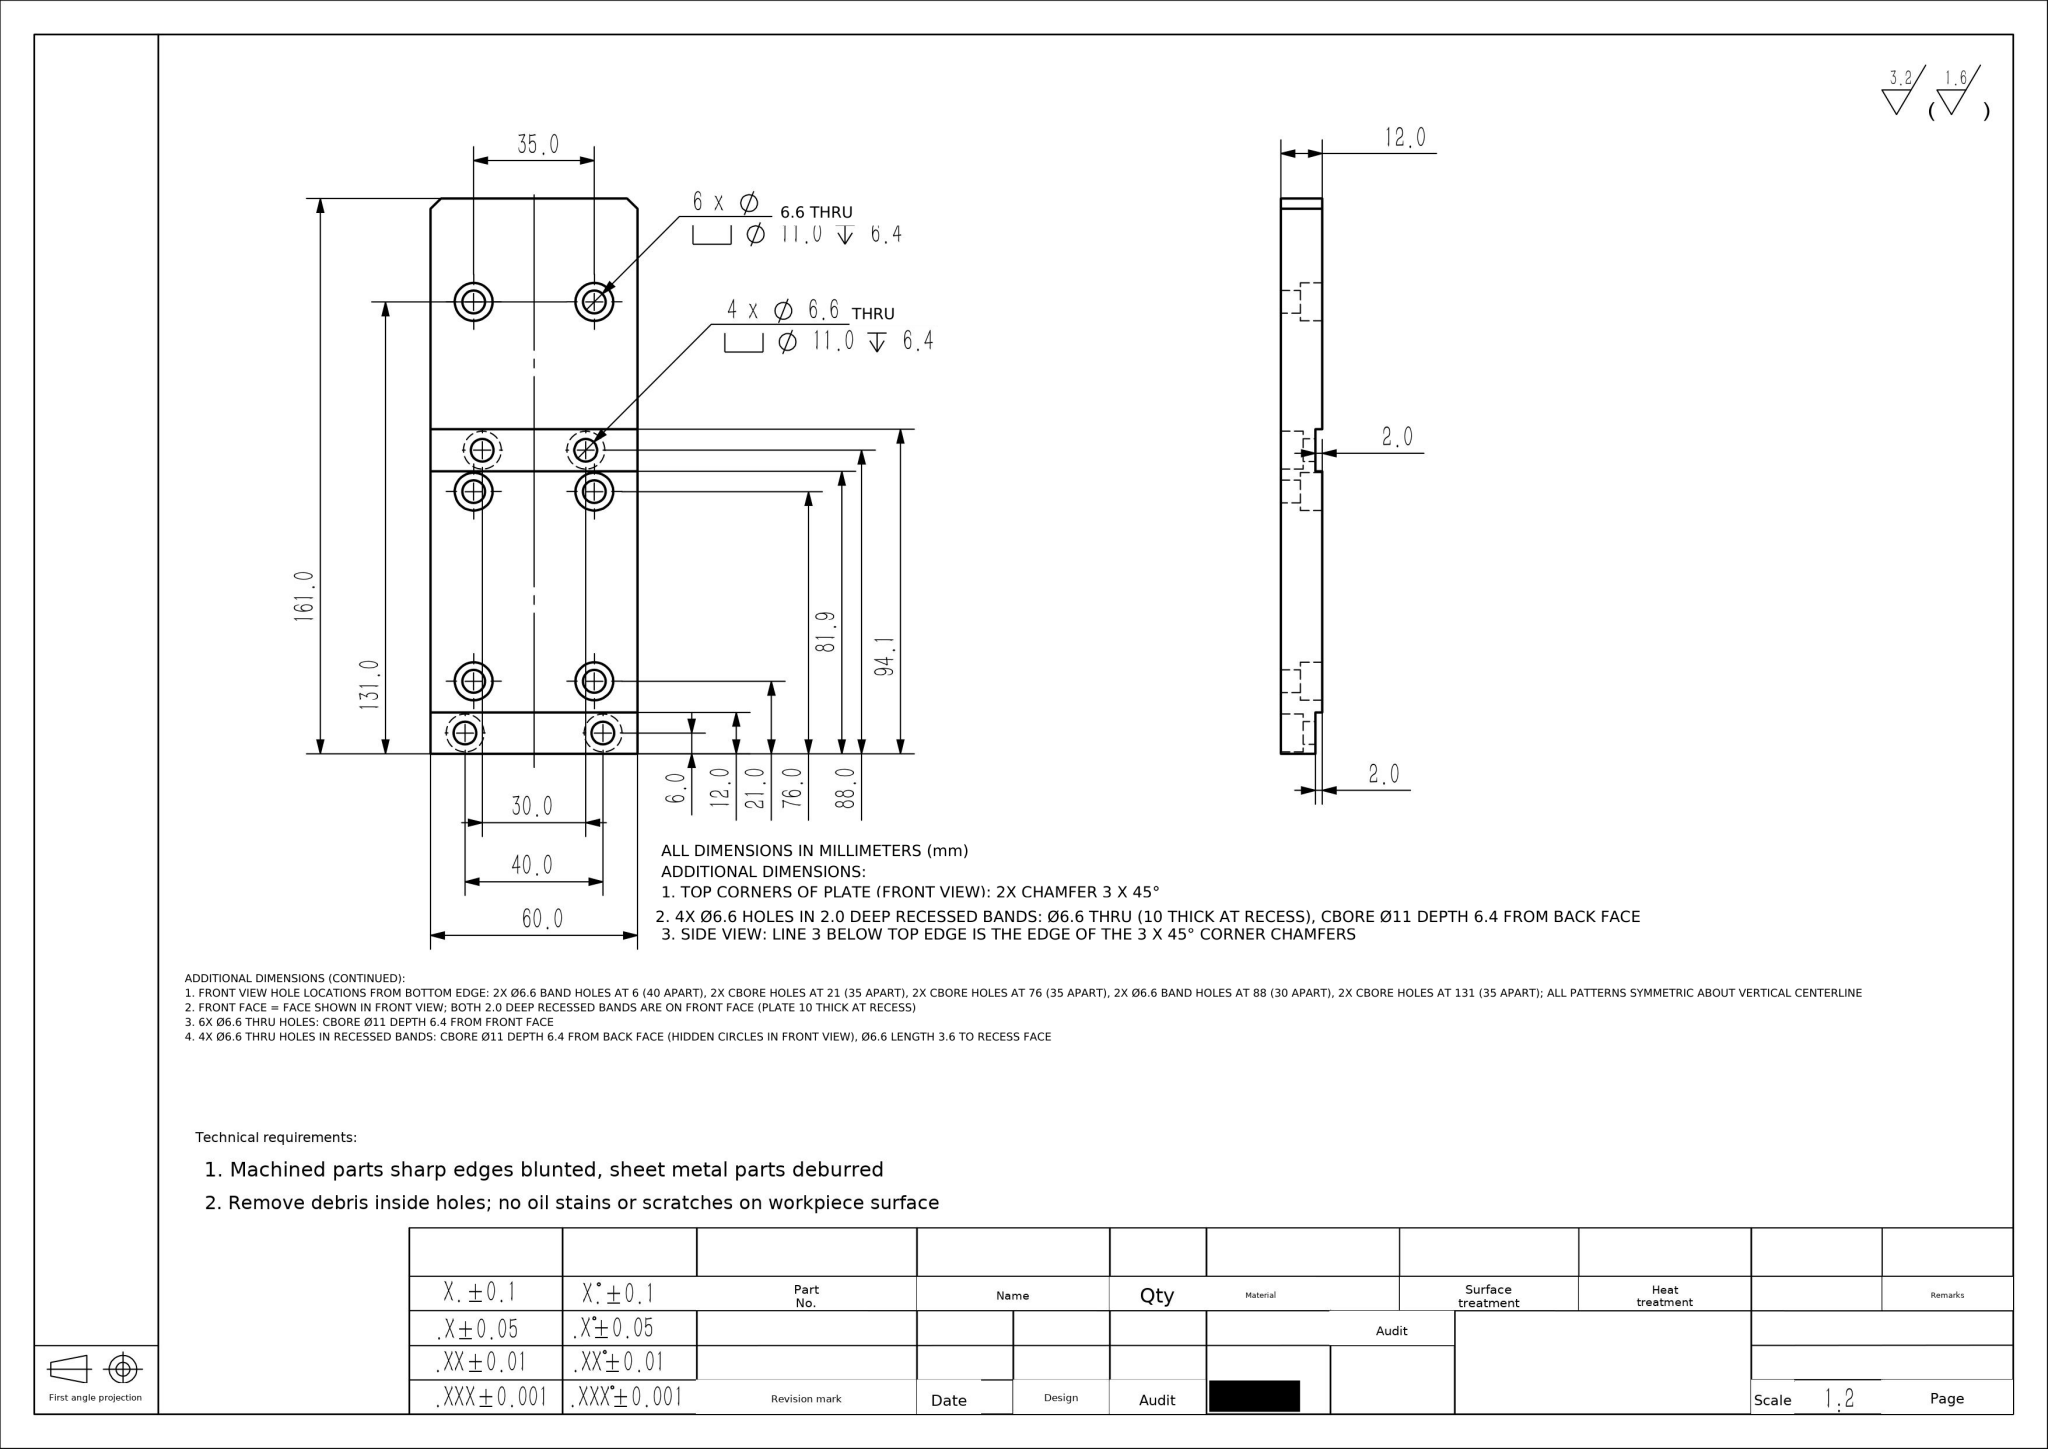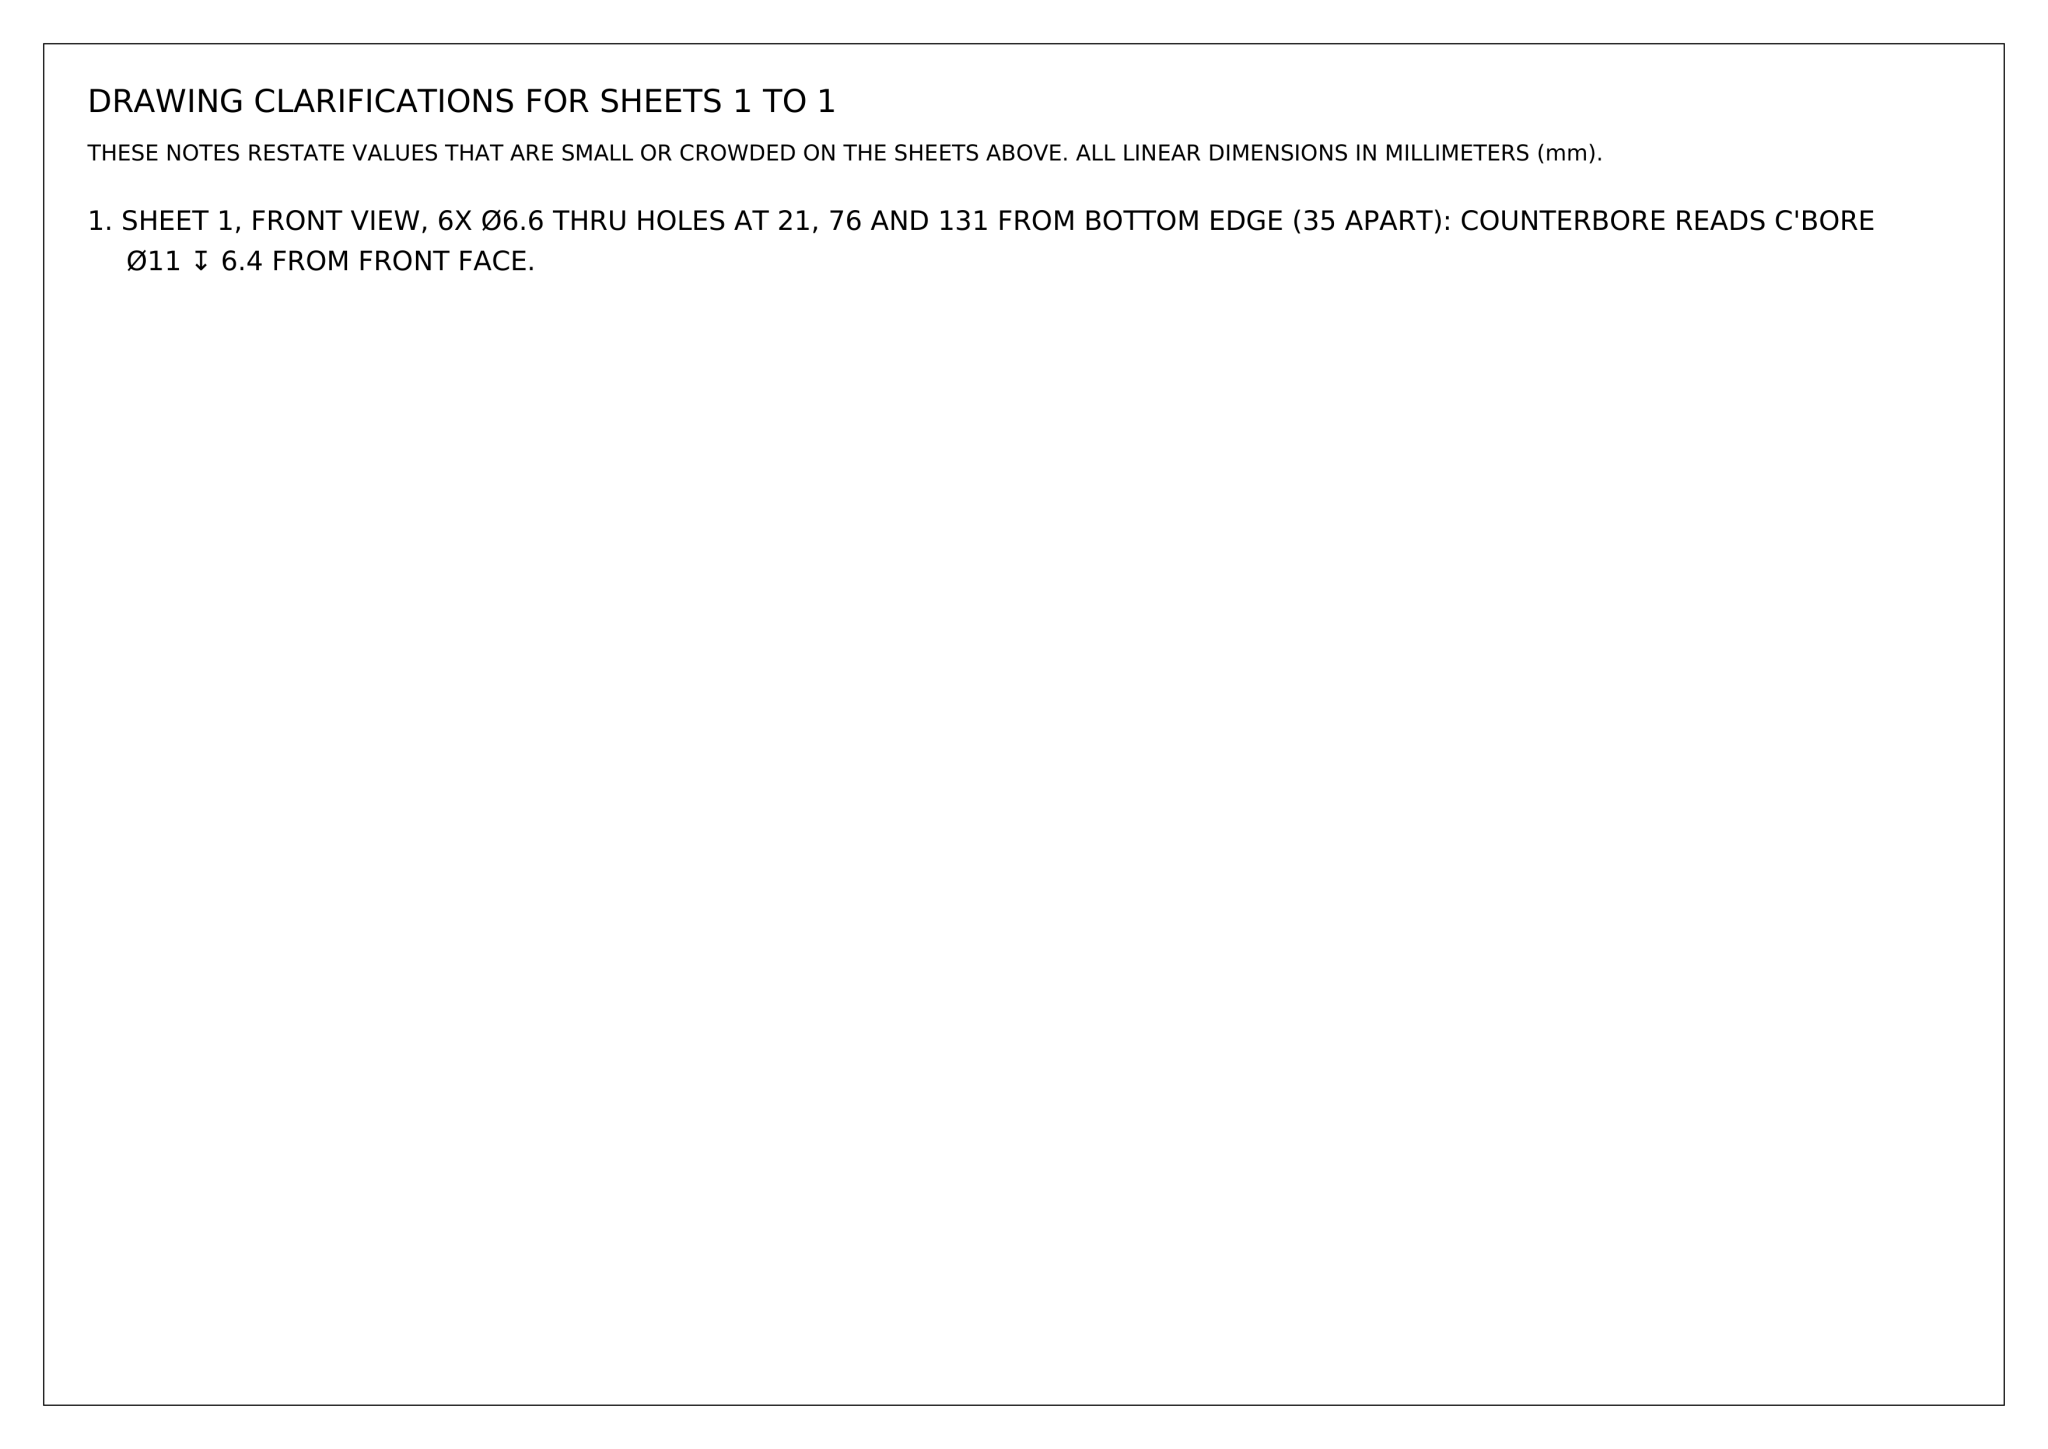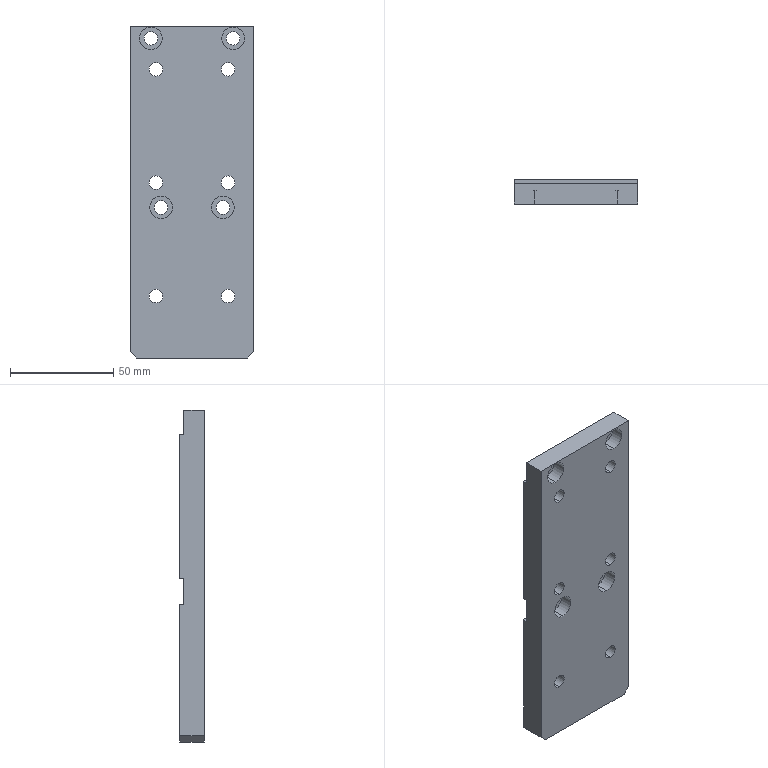Part | NX | mm | 1 solid | 64 faces | box 60 x 12 x 161 mm | volume 105184 mm3 | cylinder 40 | plane 24 | commonest cylinder face diameters 11 x20 6.6 x20